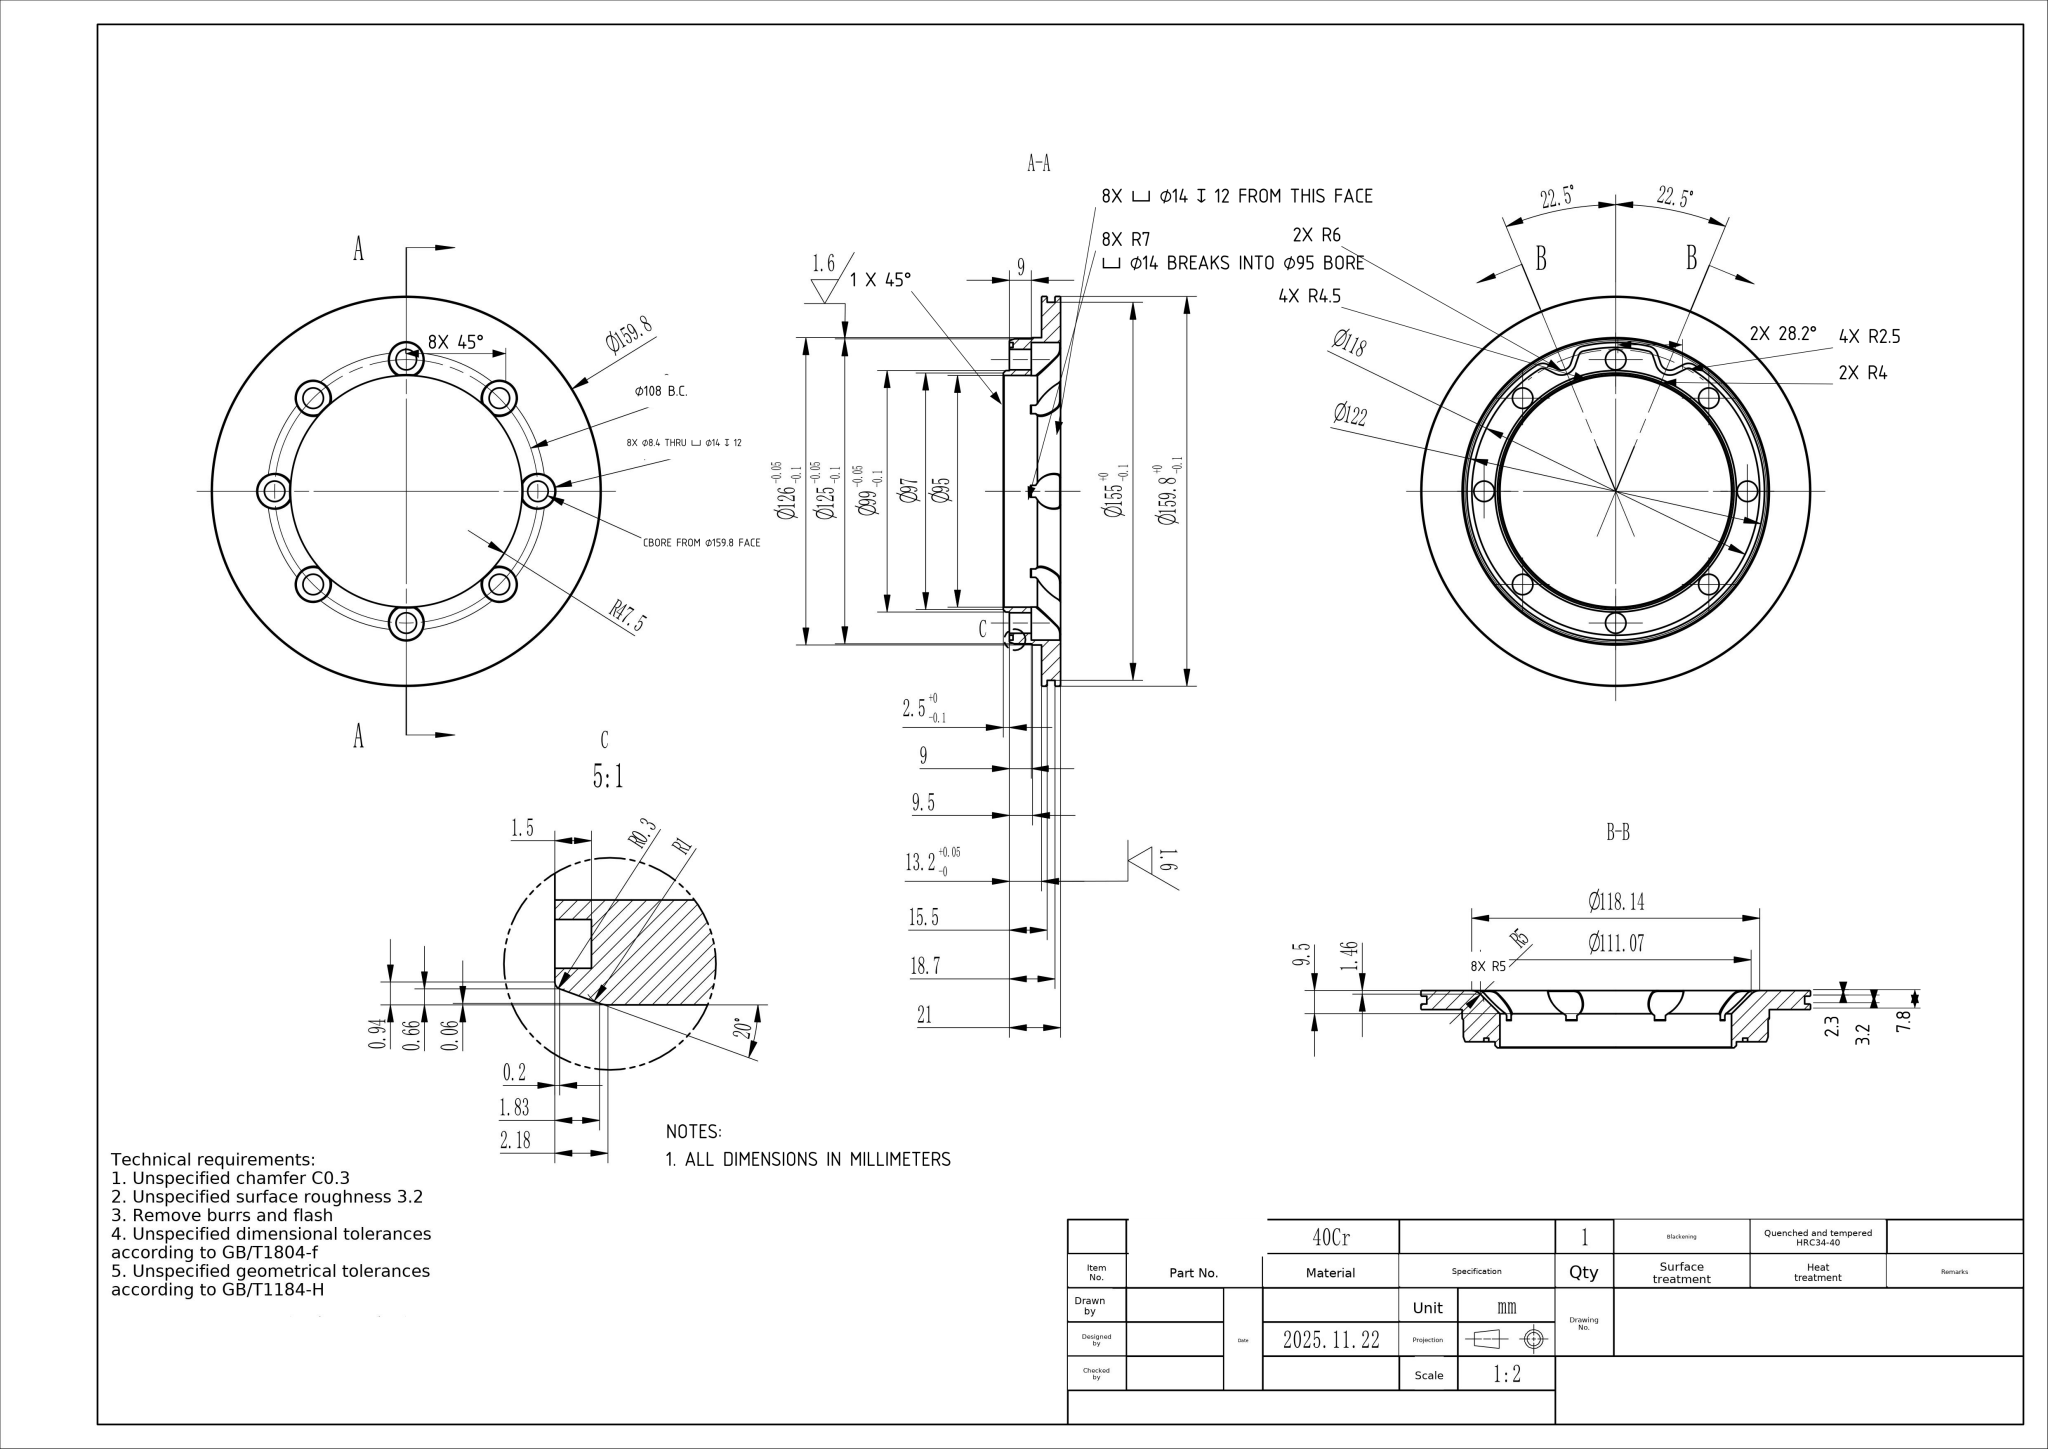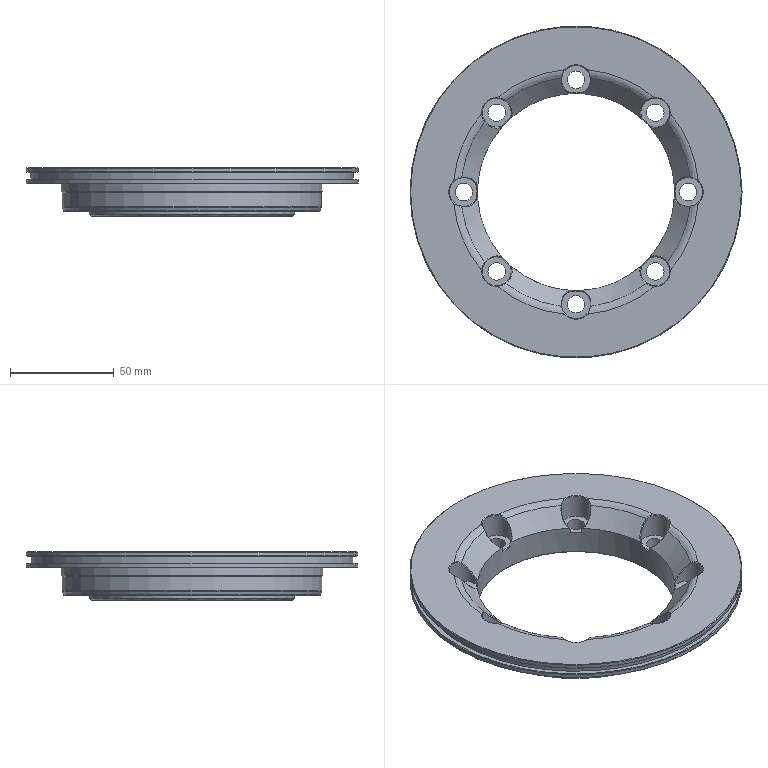Part | NX | mm | 1 solid | 137 faces | box 159.8 x 159.8 x 23.5 mm | volume 137173 mm3 | cylinder 39 | cone 32 | spline 32 | plane 24 | torus 10 | commonest cylinder face diameters 14 x8 8.4 x8 5 x4 9 x4 159.8 x2 118 x2 12 x2 8 x2